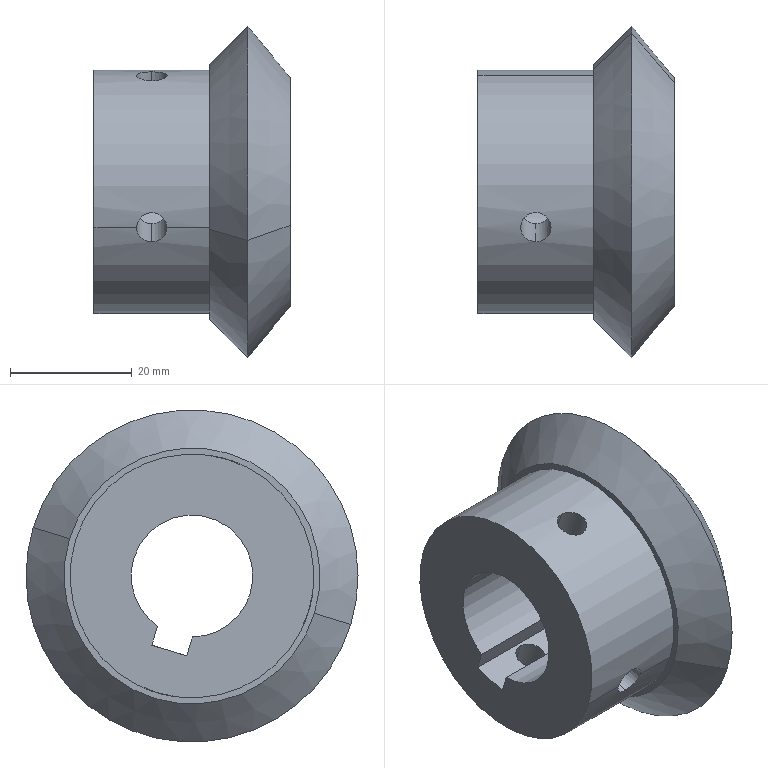Component | SolidWorks | ZL-11-12Gear-1 | 1 solid | 23 faces | box 32.19 x 54.5 x 54.5 mm | volume 33785 mm3 | cylinder 11 | cone 6 | plane 6 | commonest cylinder face diameters 5 x6 20 x3 40 x2
build123d program:
from build123d import *

# Parameters (mm, degrees)
CUT_EXTRUDE1_DEPTH = 51.211
CIRPATTERN1_COUNT  = 3
CIRPATTERN1_ANGLE  = 180


with BuildPart() as part:
    # Sketch1 → Revolve1 (revolve)
    with BuildSketch(Plane.XY, mode=Mode.PRIVATE) as revolve1_sk:
        Polygon((9.813, 15.272), (9.813, 0), (38.5, 0), (38.5, 20), (19.5, 20), (19.5, 21), (13.25, 27.25), (6.313, 18.772), align=None)
    revolve(revolve1_sk.sketch.rotate(Axis((-41.12, 0, 0), (1, 0, 0)), 90), axis=Axis((-41.12, 0, 0), (1, 0, 0)))

    # Sketch2 → Cut-Extrude1 (cut, through all)
    with BuildSketch(Plane(origin=(38.5, 0, 0), x_dir=(0, 0, -1), z_dir=(1, 0, 0))):
        with BuildLine():
            Line((-3, 12.8), (-3, 9.539))
            ThreePointArc((-3, 9.539), (0, -10), (3, 9.539))
            Line((3, 9.539), (3, 12.8))
            Line((3, 12.8), (-3, 12.8))
        make_face()
    extrude(amount=-CUT_EXTRUDE1_DEPTH, mode=Mode.SUBTRACT)

    # Sketch3 → M6 Tapped Hole1 (revolve, cut)
    with BuildSketch(Plane(origin=(29, 24, 0), x_dir=(0, 0, 1), z_dir=(1, 0, 0))):
        Polygon((0, 0), (0, 16.502), (2.5, 15), (2.5, 0), align=None)
    m6_tapped_hole1 = revolve(axis=Axis((29, 30.35, 0), (0, -1, 0)), mode=Mode.SUBTRACT)

    # CirPattern1: M6 Tapped Hole1 ×3 about axis
    cirpattern1_axis = Axis((6.313, 0, 0), (1, 0, 0))
    for i in range(1, CIRPATTERN1_COUNT):
        add(m6_tapped_hole1.rotate(cirpattern1_axis, i * CIRPATTERN1_ANGLE / (CIRPATTERN1_COUNT - 1)), mode=Mode.SUBTRACT)


solid = part.part

# Placed as in the assembly
solid = solid.moved(Location((111.165, 111.22, -0.0002338), (106.972, 0, 180)))